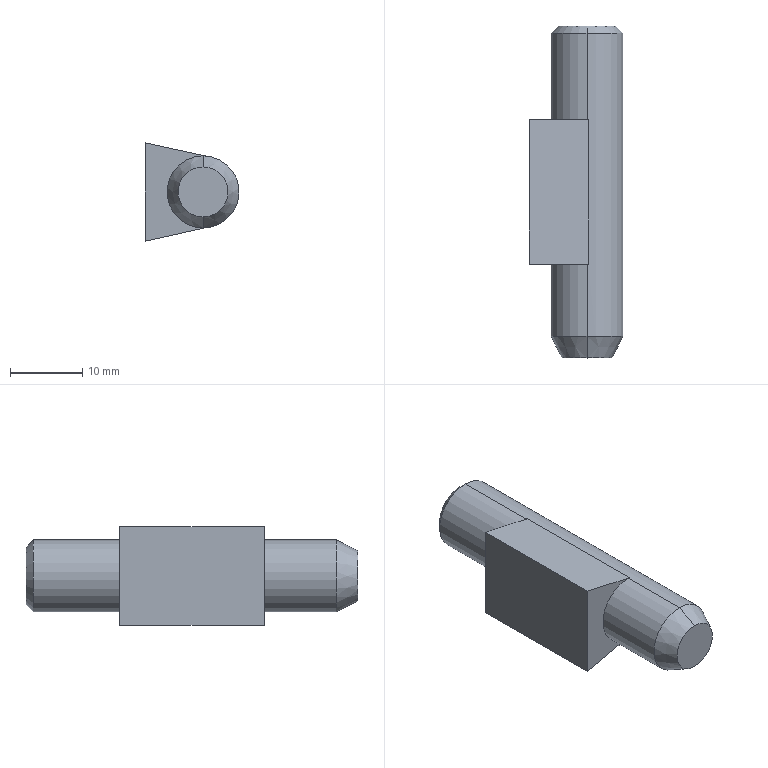Component | SolidWorks | Part21-1 | 1 solid | 20 faces | box 13.03 x 46 x 13.63 mm | volume 2575 mm3 | plane 9 | cylinder 7 | cone 4 | commonest cylinder face diameters 10 x3 8 x2 5.2 x2
STEP:
#1=COLOUR_RGB('',0.7922,0.8196,0.9333);
#2=FILL_AREA_STYLE_COLOUR('',#1);
#3=FILL_AREA_STYLE('',(#2));
#4=SURFACE_STYLE_FILL_AREA(#3);
#5=SURFACE_SIDE_STYLE('',(#4));
#6=SURFACE_STYLE_USAGE(.BOTH.,#5);
#7=PRESENTATION_STYLE_ASSIGNMENT((#6));
#8=CARTESIAN_POINT('',(6.044,10.866,-16.395));
#9=VERTEX_POINT('',#8);
#10=CARTESIAN_POINT('',(6.044,10.866,-16.08));
#11=VERTEX_POINT('',#10);
#12=CARTESIAN_POINT('',(6.044,10.866,-16.238));
#13=DIRECTION('',(0.,1.,0.));
#14=DIRECTION('',(0.,0.,-1.));
#15=AXIS2_PLACEMENT_3D('',#12,#13,#14);
#16=CIRCLE('',#15,0.1575);
#17=EDGE_CURVE('',#9,#11,#16,.T.);
#18=ORIENTED_EDGE('',*,*,#17,.F.);
#19=CARTESIAN_POINT('',(6.044,10.827,-16.434));
#20=VERTEX_POINT('',#19);
#21=CARTESIAN_POINT('',(6.044,10.866,-16.395));
#22=DIRECTION('',(-0.,-0.7071,-0.7071));
#23=VECTOR('',#22,39.37);
#24=LINE('',#21,#23);
#25=EDGE_CURVE('',#9,#20,#24,.T.);
#26=ORIENTED_EDGE('',*,*,#25,.T.);
#27=CARTESIAN_POINT('',(6.044,10.827,-16.041));
#28=VERTEX_POINT('',#27);
#29=CARTESIAN_POINT('',(6.044,10.827,-16.238));
#30=DIRECTION('',(-0.,-1.,-0.));
#31=DIRECTION('',(0.,0.,-1.));
#32=AXIS2_PLACEMENT_3D('',#29,#30,#31);
#33=CIRCLE('',#32,0.1969);
#34=EDGE_CURVE('',#28,#20,#33,.T.);
#35=ORIENTED_EDGE('',*,*,#34,.F.);
#36=CARTESIAN_POINT('',(6.044,10.866,-16.08));
#37=DIRECTION('',(-0.,-0.7071,0.7071));
#38=VECTOR('',#37,39.37);
#39=LINE('',#36,#38);
#40=EDGE_CURVE('',#11,#28,#39,.T.);
#41=ORIENTED_EDGE('',*,*,#40,.F.);
#42=EDGE_LOOP('',(#18,#26,#35,#41));
#43=FACE_OUTER_BOUND('',#42,.T.);
#44=CARTESIAN_POINT('',(6.044,10.866,-16.238));
#45=DIRECTION('',(-0.,-1.,-0.));
#46=DIRECTION('',(0.,0.,1.));
#47=AXIS2_PLACEMENT_3D('',#44,#45,#46);
#48=CONICAL_SURFACE('',#47,0.1575,0.7854);
#49=ADVANCED_FACE('',(#43),#48,.T.);
#50=CARTESIAN_POINT('',(6.044,10.748,-16.08));
#51=VERTEX_POINT('',#50);
#52=CARTESIAN_POINT('',(6.044,10.748,-16.395));
#53=VERTEX_POINT('',#52);
#54=CARTESIAN_POINT('',(6.044,10.748,-16.238));
#55=DIRECTION('',(0.,1.,0.));
#56=DIRECTION('',(0.,0.,-1.));
#57=AXIS2_PLACEMENT_3D('',#54,#55,#56);
#58=CIRCLE('',#57,0.1575);
#59=EDGE_CURVE('',#51,#53,#58,.T.);
#60=ORIENTED_EDGE('',*,*,#59,.T.);
#61=CARTESIAN_POINT('',(6.044,9.173,-16.395));
#62=VERTEX_POINT('',#61);
#63=CARTESIAN_POINT('',(6.044,10.748,-16.395));
#64=DIRECTION('',(-0.,-1.,-0.));
#65=VECTOR('',#64,39.37);
#66=LINE('',#63,#65);
#67=EDGE_CURVE('',#53,#62,#66,.T.);
#68=ORIENTED_EDGE('',*,*,#67,.T.);
#69=CARTESIAN_POINT('',(6.044,9.173,-16.08));
#70=VERTEX_POINT('',#69);
#71=CARTESIAN_POINT('',(6.044,9.173,-16.238));
#72=DIRECTION('',(0.,1.,0.));
#73=DIRECTION('',(0.,0.,-1.));
#74=AXIS2_PLACEMENT_3D('',#71,#72,#73);
#75=CIRCLE('',#74,0.1575);
#76=EDGE_CURVE('',#70,#62,#75,.T.);
#77=ORIENTED_EDGE('',*,*,#76,.F.);
#78=CARTESIAN_POINT('',(6.044,10.748,-16.08));
#79=DIRECTION('',(-0.,-1.,-0.));
#80=VECTOR('',#79,39.37);
#81=LINE('',#78,#80);
#82=EDGE_CURVE('',#51,#70,#81,.T.);
#83=ORIENTED_EDGE('',*,*,#82,.F.);
#84=EDGE_LOOP('',(#60,#68,#77,#83));
#85=FACE_OUTER_BOUND('',#84,.T.);
#86=CARTESIAN_POINT('',(6.044,10.748,-16.238));
#87=DIRECTION('',(-0.,-1.,-0.));
#88=DIRECTION('',(0.,0.,1.));
#89=AXIS2_PLACEMENT_3D('',#86,#87,#88);
#90=CYLINDRICAL_SURFACE('',#89,0.1575);
#91=ADVANCED_FACE('',(#85),#90,.F.);
#92=CARTESIAN_POINT('',(6.044,10.866,-16.135));
#93=VERTEX_POINT('',#92);
#94=CARTESIAN_POINT('',(6.044,10.866,-16.34));
#95=VERTEX_POINT('',#94);
#96=CARTESIAN_POINT('',(6.044,10.866,-16.238));
#97=DIRECTION('',(0.,1.,0.));
#98=DIRECTION('',(0.,0.,-1.));
#99=AXIS2_PLACEMENT_3D('',#96,#97,#98);
#100=CIRCLE('',#99,0.1024);
#101=EDGE_CURVE('',#93,#95,#100,.T.);
#102=ORIENTED_EDGE('',*,*,#101,.T.);
#103=CARTESIAN_POINT('',(6.044,10.748,-16.34));
#104=VERTEX_POINT('',#103);
#105=CARTESIAN_POINT('',(6.044,10.866,-16.34));
#106=DIRECTION('',(-0.,-1.,-0.));
#107=VECTOR('',#106,39.37);
#108=LINE('',#105,#107);
#109=EDGE_CURVE('',#95,#104,#108,.T.);
#110=ORIENTED_EDGE('',*,*,#109,.T.);
#111=CARTESIAN_POINT('',(6.044,10.748,-16.135));
#112=VERTEX_POINT('',#111);
#113=CARTESIAN_POINT('',(6.044,10.748,-16.238));
#114=DIRECTION('',(0.,1.,0.));
#115=DIRECTION('',(0.,0.,-1.));
#116=AXIS2_PLACEMENT_3D('',#113,#114,#115);
#117=CIRCLE('',#116,0.1024);
#118=EDGE_CURVE('',#112,#104,#117,.T.);
#119=ORIENTED_EDGE('',*,*,#118,.F.);
#120=CARTESIAN_POINT('',(6.044,10.866,-16.135));
#121=DIRECTION('',(-0.,-1.,-0.));
#122=VECTOR('',#121,39.37);
#123=LINE('',#120,#122);
#124=EDGE_CURVE('',#93,#112,#123,.T.);
#125=ORIENTED_EDGE('',*,*,#124,.F.);
#126=EDGE_LOOP('',(#102,#110,#119,#125));
#127=FACE_OUTER_BOUND('',#126,.T.);
#128=CARTESIAN_POINT('',(6.044,10.866,-16.238));
#129=DIRECTION('',(-0.,-1.,-0.));
#130=DIRECTION('',(0.,0.,1.));
#131=AXIS2_PLACEMENT_3D('',#128,#129,#130);
#132=CYLINDRICAL_SURFACE('',#131,0.1024);
#133=ADVANCED_FACE('',(#127),#132,.F.);
#134=CARTESIAN_POINT('',(6.044,9.055,-16.374));
#135=VERTEX_POINT('',#134);
#136=CARTESIAN_POINT('',(6.044,9.055,-16.101));
#137=VERTEX_POINT('',#136);
#138=CARTESIAN_POINT('',(6.044,9.055,-16.238));
#139=DIRECTION('',(-0.,-1.,-0.));
#140=DIRECTION('',(0.,0.,1.));
#141=AXIS2_PLACEMENT_3D('',#138,#139,#140);
#142=CIRCLE('',#141,0.1367);
#143=EDGE_CURVE('',#135,#137,#142,.T.);
#144=ORIENTED_EDGE('',*,*,#143,.F.);
#145=CARTESIAN_POINT('',(6.044,9.173,-16.434));
#146=VERTEX_POINT('',#145);
#147=CARTESIAN_POINT('',(6.044,9.173,-16.434));
#148=DIRECTION('',(0.,0.891,-0.454));
#149=VECTOR('',#148,39.37);
#150=LINE('',#147,#149);
#151=EDGE_CURVE('',#135,#146,#150,.T.);
#152=ORIENTED_EDGE('',*,*,#151,.T.);
#153=CARTESIAN_POINT('',(6.044,9.173,-16.041));
#154=VERTEX_POINT('',#153);
#155=CARTESIAN_POINT('',(6.044,9.173,-16.238));
#156=DIRECTION('',(-0.,-1.,-0.));
#157=DIRECTION('',(0.,0.,1.));
#158=AXIS2_PLACEMENT_3D('',#155,#156,#157);
#159=CIRCLE('',#158,0.1969);
#160=EDGE_CURVE('',#146,#154,#159,.T.);
#161=ORIENTED_EDGE('',*,*,#160,.T.);
#162=CARTESIAN_POINT('',(6.044,9.173,-16.041));
#163=DIRECTION('',(0.,0.891,0.454));
#164=VECTOR('',#163,39.37);
#165=LINE('',#162,#164);
#166=EDGE_CURVE('',#137,#154,#165,.T.);
#167=ORIENTED_EDGE('',*,*,#166,.F.);
#168=EDGE_LOOP('',(#144,#152,#161,#167));
#169=FACE_OUTER_BOUND('',#168,.T.);
#170=CARTESIAN_POINT('',(6.044,9.173,-16.238));
#171=DIRECTION('',(0.,1.,0.));
#172=DIRECTION('',(0.,0.,1.));
#173=AXIS2_PLACEMENT_3D('',#170,#171,#172);
#174=CONICAL_SURFACE('',#173,0.1969,0.4712);
#175=ADVANCED_FACE('',(#169),#174,.T.);
#176=ORIENTED_EDGE('',*,*,#34,.T.);
#177=CARTESIAN_POINT('',(6.044,10.354,-16.434));
#178=VERTEX_POINT('',#177);
#179=CARTESIAN_POINT('',(6.044,10.748,-16.434));
#180=DIRECTION('',(-0.,-1.,-0.));
#181=VECTOR('',#180,39.37);
#182=LINE('',#179,#181);
#183=EDGE_CURVE('',#20,#178,#182,.T.);
#184=ORIENTED_EDGE('',*,*,#183,.T.);
#185=CARTESIAN_POINT('',(6.044,10.354,-16.041));
#186=VERTEX_POINT('',#185);
#187=CARTESIAN_POINT('',(6.044,10.354,-16.238));
#188=DIRECTION('',(0.,1.,0.));
#189=DIRECTION('',(0.,0.,1.));
#190=AXIS2_PLACEMENT_3D('',#187,#188,#189);
#191=CIRCLE('',#190,0.1969);
#192=EDGE_CURVE('',#178,#186,#191,.T.);
#193=ORIENTED_EDGE('',*,*,#192,.T.);
#194=CARTESIAN_POINT('',(6.044,10.748,-16.041));
#195=DIRECTION('',(-0.,-1.,-0.));
#196=VECTOR('',#195,39.37);
#197=LINE('',#194,#196);
#198=EDGE_CURVE('',#28,#186,#197,.T.);
#199=ORIENTED_EDGE('',*,*,#198,.F.);
#200=EDGE_LOOP('',(#176,#184,#193,#199));
#201=FACE_OUTER_BOUND('',#200,.T.);
#202=CARTESIAN_POINT('',(6.044,10.748,-16.238));
#203=DIRECTION('',(-0.,-1.,-0.));
#204=DIRECTION('',(0.,0.,1.));
#205=AXIS2_PLACEMENT_3D('',#202,#203,#204);
#206=CYLINDRICAL_SURFACE('',#205,0.1969);
#207=ADVANCED_FACE('',(#201),#206,.T.);
#208=CARTESIAN_POINT('',(6.044,9.567,-16.434));
#209=VERTEX_POINT('',#208);
#210=CARTESIAN_POINT('',(6.044,9.567,-16.041));
#211=VERTEX_POINT('',#210);
#212=CARTESIAN_POINT('',(6.044,9.567,-16.238));
#213=DIRECTION('',(0.,1.,0.));
#214=DIRECTION('',(0.,0.,1.));
#215=AXIS2_PLACEMENT_3D('',#212,#213,#214);
#216=CIRCLE('',#215,0.1969);
#217=EDGE_CURVE('',#209,#211,#216,.T.);
#218=ORIENTED_EDGE('',*,*,#217,.F.);
#219=CARTESIAN_POINT('',(6.044,10.748,-16.434));
#220=DIRECTION('',(-0.,-1.,-0.));
#221=VECTOR('',#220,39.37);
#222=LINE('',#219,#221);
#223=EDGE_CURVE('',#209,#146,#222,.T.);
#224=ORIENTED_EDGE('',*,*,#223,.T.);
#225=CARTESIAN_POINT('',(6.044,9.173,-16.238));
#226=DIRECTION('',(-0.,-1.,-0.));
#227=DIRECTION('',(0.,0.,1.));
#228=AXIS2_PLACEMENT_3D('',#225,#226,#227);
#229=CIRCLE('',#228,0.1969);
#230=EDGE_CURVE('',#154,#146,#229,.T.);
#231=ORIENTED_EDGE('',*,*,#230,.F.);
#232=CARTESIAN_POINT('',(6.044,10.748,-16.041));
#233=DIRECTION('',(-0.,-1.,-0.));
#234=VECTOR('',#233,39.37);
#235=LINE('',#232,#234);
#236=EDGE_CURVE('',#211,#154,#235,.T.);
#237=ORIENTED_EDGE('',*,*,#236,.F.);
#238=EDGE_LOOP('',(#218,#224,#231,#237));
#239=FACE_OUTER_BOUND('',#238,.T.);
#240=CARTESIAN_POINT('',(6.044,10.748,-16.238));
#241=DIRECTION('',(-0.,-1.,-0.));
#242=DIRECTION('',(0.,0.,1.));
#243=AXIS2_PLACEMENT_3D('',#240,#241,#242);
#244=CYLINDRICAL_SURFACE('',#243,0.1969);
#245=ADVANCED_FACE('',(#239),#244,.T.);
#246=ORIENTED_EDGE('',*,*,#183,.F.);
#247=CARTESIAN_POINT('',(6.044,10.827,-16.238));
#248=DIRECTION('',(-0.,-1.,-0.));
#249=DIRECTION('',(0.,0.,-1.));
#250=AXIS2_PLACEMENT_3D('',#247,#248,#249);
#251=CIRCLE('',#250,0.1969);
#252=EDGE_CURVE('',#20,#28,#251,.T.);
#253=ORIENTED_EDGE('',*,*,#252,.T.);
#254=ORIENTED_EDGE('',*,*,#198,.T.);
#255=CARTESIAN_POINT('',(6.051,10.354,-16.041));
#256=VERTEX_POINT('',#255);
#257=CARTESIAN_POINT('',(6.044,10.354,-16.238));
#258=DIRECTION('',(0.,1.,0.));
#259=DIRECTION('',(0.,0.,1.));
#260=AXIS2_PLACEMENT_3D('',#257,#258,#259);
#261=CIRCLE('',#260,0.1969);
#262=EDGE_CURVE('',#186,#256,#261,.T.);
#263=ORIENTED_EDGE('',*,*,#262,.T.);
#264=CARTESIAN_POINT('',(6.051,9.567,-16.041));
#265=VERTEX_POINT('',#264);
#266=CARTESIAN_POINT('',(6.051,9.567,-16.041));
#267=DIRECTION('',(0.,1.,0.));
#268=VECTOR('',#267,39.37);
#269=LINE('',#266,#268);
#270=EDGE_CURVE('',#265,#256,#269,.T.);
#271=ORIENTED_EDGE('',*,*,#270,.F.);
#272=CARTESIAN_POINT('',(6.044,9.567,-16.238));
#273=DIRECTION('',(0.,1.,0.));
#274=DIRECTION('',(0.,0.,1.));
#275=AXIS2_PLACEMENT_3D('',#272,#273,#274);
#276=CIRCLE('',#275,0.1969);
#277=EDGE_CURVE('',#211,#265,#276,.T.);
#278=ORIENTED_EDGE('',*,*,#277,.F.);
#279=ORIENTED_EDGE('',*,*,#236,.T.);
#280=ORIENTED_EDGE('',*,*,#160,.F.);
#281=ORIENTED_EDGE('',*,*,#223,.F.);
#282=CARTESIAN_POINT('',(6.051,9.567,-16.434));
#283=VERTEX_POINT('',#282);
#284=CARTESIAN_POINT('',(6.044,9.567,-16.238));
#285=DIRECTION('',(0.,1.,0.));
#286=DIRECTION('',(0.,0.,1.));
#287=AXIS2_PLACEMENT_3D('',#284,#285,#286);
#288=CIRCLE('',#287,0.1969);
#289=EDGE_CURVE('',#283,#209,#288,.T.);
#290=ORIENTED_EDGE('',*,*,#289,.F.);
#291=CARTESIAN_POINT('',(6.051,10.354,-16.434));
#292=VERTEX_POINT('',#291);
#293=CARTESIAN_POINT('',(6.051,9.567,-16.434));
#294=DIRECTION('',(0.,1.,0.));
#295=VECTOR('',#294,39.37);
#296=LINE('',#293,#295);
#297=EDGE_CURVE('',#283,#292,#296,.T.);
#298=ORIENTED_EDGE('',*,*,#297,.T.);
#299=CARTESIAN_POINT('',(6.044,10.354,-16.238));
#300=DIRECTION('',(0.,1.,0.));
#301=DIRECTION('',(0.,0.,1.));
#302=AXIS2_PLACEMENT_3D('',#299,#300,#301);
#303=CIRCLE('',#302,0.1969);
#304=EDGE_CURVE('',#292,#178,#303,.T.);
#305=ORIENTED_EDGE('',*,*,#304,.T.);
#306=EDGE_LOOP('',(#246,#253,#254,#263,#271,#278,#279,#280,#281,#290,#298,#305));
#307=FACE_OUTER_BOUND('',#306,.T.);
#308=CARTESIAN_POINT('',(6.044,10.748,-16.238));
#309=DIRECTION('',(-0.,-1.,-0.));
#310=DIRECTION('',(0.,0.,1.));
#311=AXIS2_PLACEMENT_3D('',#308,#309,#310);
#312=CYLINDRICAL_SURFACE('',#311,0.1969);
#313=ADVANCED_FACE('',(#307),#312,.T.);
#314=ORIENTED_EDGE('',*,*,#151,.F.);
#315=CARTESIAN_POINT('',(6.044,9.055,-16.238));
#316=DIRECTION('',(-0.,-1.,-0.));
#317=DIRECTION('',(0.,0.,1.));
#318=AXIS2_PLACEMENT_3D('',#315,#316,#317);
#319=CIRCLE('',#318,0.1367);
#320=EDGE_CURVE('',#137,#135,#319,.T.);
#321=ORIENTED_EDGE('',*,*,#320,.F.);
#322=ORIENTED_EDGE('',*,*,#166,.T.);
#323=ORIENTED_EDGE('',*,*,#230,.T.);
#324=EDGE_LOOP('',(#314,#321,#322,#323));
#325=FACE_OUTER_BOUND('',#324,.T.);
#326=CARTESIAN_POINT('',(6.044,9.173,-16.238));
#327=DIRECTION('',(0.,1.,0.));
#328=DIRECTION('',(0.,0.,1.));
#329=AXIS2_PLACEMENT_3D('',#326,#327,#328);
#330=CONICAL_SURFACE('',#329,0.1969,0.4712);
#331=ADVANCED_FACE('',(#325),#330,.T.);
#332=ORIENTED_EDGE('',*,*,#320,.T.);
#333=ORIENTED_EDGE('',*,*,#143,.T.);
#334=EDGE_LOOP('',(#332,#333));
#335=FACE_OUTER_BOUND('',#334,.T.);
#336=CARTESIAN_POINT('',(6.044,9.055,-16.238));
#337=DIRECTION('',(-0.,-1.,-0.));
#338=DIRECTION('',(0.,-0.,1.));
#339=AXIS2_PLACEMENT_3D('',#336,#337,#338);
#340=PLANE('',#339);
#341=ADVANCED_FACE('',(#335),#340,.T.);
#342=ORIENTED_EDGE('',*,*,#270,.T.);
#343=CARTESIAN_POINT('',(5.728,10.354,-15.97));
#344=VERTEX_POINT('',#343);
#345=CARTESIAN_POINT('',(5.728,10.354,-15.97));
#346=DIRECTION('',(-0.9766,0.,0.2149));
#347=VECTOR('',#346,39.37);
#348=LINE('',#345,#347);
#349=EDGE_CURVE('',#256,#344,#348,.T.);
#350=ORIENTED_EDGE('',*,*,#349,.T.);
#351=CARTESIAN_POINT('',(5.728,9.567,-15.97));
#352=VERTEX_POINT('',#351);
#353=CARTESIAN_POINT('',(5.728,9.567,-15.97));
#354=DIRECTION('',(0.,1.,0.));
#355=VECTOR('',#354,39.37);
#356=LINE('',#353,#355);
#357=EDGE_CURVE('',#352,#344,#356,.T.);
#358=ORIENTED_EDGE('',*,*,#357,.F.);
#359=CARTESIAN_POINT('',(5.728,9.567,-15.97));
#360=DIRECTION('',(-0.9766,0.,0.2149));
#361=VECTOR('',#360,39.37);
#362=LINE('',#359,#361);
#363=EDGE_CURVE('',#265,#352,#362,.T.);
#364=ORIENTED_EDGE('',*,*,#363,.F.);
#365=EDGE_LOOP('',(#342,#350,#358,#364));
#366=FACE_OUTER_BOUND('',#365,.T.);
#367=CARTESIAN_POINT('',(5.728,9.567,-15.97));
#368=DIRECTION('',(-0.2149,0.,-0.9766));
#369=DIRECTION('',(-0.9766,0.,0.2149));
#370=AXIS2_PLACEMENT_3D('',#367,#368,#369);
#371=PLANE('',#370);
#372=ADVANCED_FACE('',(#366),#371,.F.);
#373=ORIENTED_EDGE('',*,*,#357,.T.);
#374=CARTESIAN_POINT('',(5.728,10.354,-16.506));
#375=VERTEX_POINT('',#374);
#376=CARTESIAN_POINT('',(5.728,10.354,-16.506));
#377=DIRECTION('',(-0.,0.,-1.));
#378=VECTOR('',#377,39.37);
#379=LINE('',#376,#378);
#380=EDGE_CURVE('',#344,#375,#379,.T.);
#381=ORIENTED_EDGE('',*,*,#380,.T.);
#382=CARTESIAN_POINT('',(5.728,9.567,-16.506));
#383=VERTEX_POINT('',#382);
#384=CARTESIAN_POINT('',(5.728,9.567,-16.506));
#385=DIRECTION('',(0.,1.,0.));
#386=VECTOR('',#385,39.37);
#387=LINE('',#384,#386);
#388=EDGE_CURVE('',#383,#375,#387,.T.);
#389=ORIENTED_EDGE('',*,*,#388,.F.);
#390=CARTESIAN_POINT('',(5.728,9.567,-16.506));
#391=DIRECTION('',(-0.,0.,-1.));
#392=VECTOR('',#391,39.37);
#393=LINE('',#390,#392);
#394=EDGE_CURVE('',#352,#383,#393,.T.);
#395=ORIENTED_EDGE('',*,*,#394,.F.);
#396=EDGE_LOOP('',(#373,#381,#389,#395));
#397=FACE_OUTER_BOUND('',#396,.T.);
#398=CARTESIAN_POINT('',(5.728,9.567,-16.506));
#399=DIRECTION('',(1.,-0.,-0.));
#400=DIRECTION('',(-0.,-1.,-0.));
#401=AXIS2_PLACEMENT_3D('',#398,#399,#400);
#402=PLANE('',#401);
#403=ADVANCED_FACE('',(#397),#402,.F.);
#404=ORIENTED_EDGE('',*,*,#388,.T.);
#405=CARTESIAN_POINT('',(6.051,10.354,-16.434));
#406=DIRECTION('',(0.9759,-0.,0.218));
#407=VECTOR('',#406,39.37);
#408=LINE('',#405,#407);
#409=EDGE_CURVE('',#375,#292,#408,.T.);
#410=ORIENTED_EDGE('',*,*,#409,.T.);
#411=ORIENTED_EDGE('',*,*,#297,.F.);
#412=CARTESIAN_POINT('',(6.051,9.567,-16.434));
#413=DIRECTION('',(0.9759,-0.,0.218));
#414=VECTOR('',#413,39.37);
#415=LINE('',#412,#414);
#416=EDGE_CURVE('',#383,#283,#415,.T.);
#417=ORIENTED_EDGE('',*,*,#416,.F.);
#418=EDGE_LOOP('',(#404,#410,#411,#417));
#419=FACE_OUTER_BOUND('',#418,.T.);
#420=CARTESIAN_POINT('',(6.051,9.567,-16.434));
#421=DIRECTION('',(-0.218,0.,0.9759));
#422=DIRECTION('',(0.9759,-0.,0.218));
#423=AXIS2_PLACEMENT_3D('',#420,#421,#422);
#424=PLANE('',#423);
#425=ADVANCED_FACE('',(#419),#424,.F.);
#426=ORIENTED_EDGE('',*,*,#289,.T.);
#427=ORIENTED_EDGE('',*,*,#217,.T.);
#428=ORIENTED_EDGE('',*,*,#277,.T.);
#429=ORIENTED_EDGE('',*,*,#363,.T.);
#430=ORIENTED_EDGE('',*,*,#394,.T.);
#431=ORIENTED_EDGE('',*,*,#416,.T.);
#432=EDGE_LOOP('',(#426,#427,#428,#429,#430,#431));
#433=FACE_OUTER_BOUND('',#432,.T.);
#434=CARTESIAN_POINT('',(6.044,9.567,-16.238));
#435=DIRECTION('',(-0.,-1.,-0.));
#436=DIRECTION('',(0.,-0.,1.));
#437=AXIS2_PLACEMENT_3D('',#434,#435,#436);
#438=PLANE('',#437);
#439=ADVANCED_FACE('',(#433),#438,.T.);
#440=ORIENTED_EDGE('',*,*,#304,.F.);
#441=ORIENTED_EDGE('',*,*,#409,.F.);
#442=ORIENTED_EDGE('',*,*,#380,.F.);
#443=ORIENTED_EDGE('',*,*,#349,.F.);
#444=ORIENTED_EDGE('',*,*,#262,.F.);
#445=ORIENTED_EDGE('',*,*,#192,.F.);
#446=EDGE_LOOP('',(#440,#441,#442,#443,#444,#445));
#447=FACE_OUTER_BOUND('',#446,.T.);
#448=CARTESIAN_POINT('',(6.044,10.354,-16.238));
#449=DIRECTION('',(-0.,-1.,-0.));
#450=DIRECTION('',(0.,-0.,1.));
#451=AXIS2_PLACEMENT_3D('',#448,#449,#450);
#452=PLANE('',#451);
#453=ADVANCED_FACE('',(#447),#452,.F.);
#454=ORIENTED_EDGE('',*,*,#118,.T.);
#455=CARTESIAN_POINT('',(6.044,10.748,-16.238));
#456=DIRECTION('',(0.,1.,0.));
#457=DIRECTION('',(0.,0.,-1.));
#458=AXIS2_PLACEMENT_3D('',#455,#456,#457);
#459=CIRCLE('',#458,0.1024);
#460=EDGE_CURVE('',#104,#112,#459,.T.);
#461=ORIENTED_EDGE('',*,*,#460,.T.);
#462=EDGE_LOOP('',(#454,#461));
#463=FACE_BOUND('',#462,.T.);
#464=ORIENTED_EDGE('',*,*,#59,.F.);
#465=CARTESIAN_POINT('',(6.044,10.748,-16.238));
#466=DIRECTION('',(0.,1.,0.));
#467=DIRECTION('',(0.,0.,-1.));
#468=AXIS2_PLACEMENT_3D('',#465,#466,#467);
#469=CIRCLE('',#468,0.1575);
#470=EDGE_CURVE('',#53,#51,#469,.T.);
#471=ORIENTED_EDGE('',*,*,#470,.F.);
#472=EDGE_LOOP('',(#464,#471));
#473=FACE_OUTER_BOUND('',#472,.T.);
#474=CARTESIAN_POINT('',(6.044,10.748,-16.238));
#475=DIRECTION('',(0.,1.,0.));
#476=DIRECTION('',(-0.,0.,-1.));
#477=AXIS2_PLACEMENT_3D('',#474,#475,#476);
#478=PLANE('',#477);
#479=ADVANCED_FACE('',(#463,#473),#478,.F.);
#480=CARTESIAN_POINT('',(6.044,10.866,-16.238));
#481=DIRECTION('',(0.,1.,0.));
#482=DIRECTION('',(0.,0.,-1.));
#483=AXIS2_PLACEMENT_3D('',#480,#481,#482);
#484=CIRCLE('',#483,0.1575);
#485=EDGE_CURVE('',#11,#9,#484,.T.);
#486=ORIENTED_EDGE('',*,*,#485,.T.);
#487=ORIENTED_EDGE('',*,*,#17,.T.);
#488=EDGE_LOOP('',(#486,#487));
#489=FACE_OUTER_BOUND('',#488,.T.);
#490=ORIENTED_EDGE('',*,*,#101,.F.);
#491=CARTESIAN_POINT('',(6.044,10.866,-16.238));
#492=DIRECTION('',(0.,1.,0.));
#493=DIRECTION('',(0.,0.,-1.));
#494=AXIS2_PLACEMENT_3D('',#491,#492,#493);
#495=CIRCLE('',#494,0.1024);
#496=EDGE_CURVE('',#95,#93,#495,.T.);
#497=ORIENTED_EDGE('',*,*,#496,.F.);
#498=EDGE_LOOP('',(#490,#497));
#499=FACE_BOUND('',#498,.T.);
#500=CARTESIAN_POINT('',(6.044,10.866,-16.238));
#501=DIRECTION('',(0.,1.,0.));
#502=DIRECTION('',(-0.,0.,-1.));
#503=AXIS2_PLACEMENT_3D('',#500,#501,#502);
#504=PLANE('',#503);
#505=ADVANCED_FACE('',(#489,#499),#504,.T.);
#506=ORIENTED_EDGE('',*,*,#109,.F.);
#507=ORIENTED_EDGE('',*,*,#496,.T.);
#508=ORIENTED_EDGE('',*,*,#124,.T.);
#509=ORIENTED_EDGE('',*,*,#460,.F.);
#510=EDGE_LOOP('',(#506,#507,#508,#509));
#511=FACE_OUTER_BOUND('',#510,.T.);
#512=CARTESIAN_POINT('',(6.044,10.866,-16.238));
#513=DIRECTION('',(-0.,-1.,-0.));
#514=DIRECTION('',(0.,0.,1.));
#515=AXIS2_PLACEMENT_3D('',#512,#513,#514);
#516=CYLINDRICAL_SURFACE('',#515,0.1024);
#517=ADVANCED_FACE('',(#511),#516,.F.);
#518=ORIENTED_EDGE('',*,*,#76,.T.);
#519=CARTESIAN_POINT('',(6.044,9.173,-16.238));
#520=DIRECTION('',(0.,1.,0.));
#521=DIRECTION('',(0.,0.,-1.));
#522=AXIS2_PLACEMENT_3D('',#519,#520,#521);
#523=CIRCLE('',#522,0.1575);
#524=EDGE_CURVE('',#62,#70,#523,.T.);
#525=ORIENTED_EDGE('',*,*,#524,.T.);
#526=EDGE_LOOP('',(#518,#525));
#527=FACE_OUTER_BOUND('',#526,.T.);
#528=CARTESIAN_POINT('',(6.044,9.173,-16.238));
#529=DIRECTION('',(-0.,-1.,-0.));
#530=DIRECTION('',(0.,-0.,1.));
#531=AXIS2_PLACEMENT_3D('',#528,#529,#530);
#532=PLANE('',#531);
#533=ADVANCED_FACE('',(#527),#532,.F.);
#534=ORIENTED_EDGE('',*,*,#67,.F.);
#535=ORIENTED_EDGE('',*,*,#470,.T.);
#536=ORIENTED_EDGE('',*,*,#82,.T.);
#537=ORIENTED_EDGE('',*,*,#524,.F.);
#538=EDGE_LOOP('',(#534,#535,#536,#537));
#539=FACE_OUTER_BOUND('',#538,.T.);
#540=CARTESIAN_POINT('',(6.044,10.748,-16.238));
#541=DIRECTION('',(-0.,-1.,-0.));
#542=DIRECTION('',(0.,0.,1.));
#543=AXIS2_PLACEMENT_3D('',#540,#541,#542);
#544=CYLINDRICAL_SURFACE('',#543,0.1575);
#545=ADVANCED_FACE('',(#539),#544,.F.);
#546=ORIENTED_EDGE('',*,*,#25,.F.);
#547=ORIENTED_EDGE('',*,*,#485,.F.);
#548=ORIENTED_EDGE('',*,*,#40,.T.);
#549=ORIENTED_EDGE('',*,*,#252,.F.);
#550=EDGE_LOOP('',(#546,#547,#548,#549));
#551=FACE_OUTER_BOUND('',#550,.T.);
#552=CARTESIAN_POINT('',(6.044,10.866,-16.238));
#553=DIRECTION('',(-0.,-1.,-0.));
#554=DIRECTION('',(0.,0.,1.));
#555=AXIS2_PLACEMENT_3D('',#552,#553,#554);
#556=CONICAL_SURFACE('',#555,0.1575,0.7854);
#557=ADVANCED_FACE('',(#551),#556,.T.);
#558=CLOSED_SHELL('',(#49,#91,#133,#175,#207,#245,#313,#331,#341,#372,#403,#425,#439,#453,#479,#505,#517,#533,#545,#557));
#559=MANIFOLD_SOLID_BREP('',#558);
#560=STYLED_ITEM('',(#7),#559);
#561=(LENGTH_UNIT()NAMED_UNIT(*)SI_UNIT($,.METRE.));
#562=LENGTH_MEASURE_WITH_UNIT(LENGTH_MEASURE(0.0254),#561);
#563=DIMENSIONAL_EXPONENTS(1.,0.,0.,0.,0.,0.,0.);
#564=(CONVERSION_BASED_UNIT('',#562)LENGTH_UNIT()NAMED_UNIT(#563));
#565=UNCERTAINTY_MEASURE_WITH_UNIT(LENGTH_MEASURE(0.00001),#564,'','');
#566=(NAMED_UNIT(*)PLANE_ANGLE_UNIT()SI_UNIT($,.RADIAN.));
#567=(NAMED_UNIT(*)SI_UNIT($,.STERADIAN.)SOLID_ANGLE_UNIT());
#568=(GEOMETRIC_REPRESENTATION_CONTEXT(3)GLOBAL_UNCERTAINTY_ASSIGNED_CONTEXT((#565))GLOBAL_UNIT_ASSIGNED_CONTEXT((#564,#566,#567))REPRESENTATION_CONTEXT('',''));
#569=MECHANICAL_DESIGN_GEOMETRIC_PRESENTATION_REPRESENTATION('',(#560),#568);
#570=CARTESIAN_POINT('',(0.,0.,0.));
#571=DIRECTION('',(0.,0.,1.));
#572=DIRECTION('',(1.,0.,0.));
#573=AXIS2_PLACEMENT_3D('',#570,#571,#572);
#574=(LENGTH_UNIT()NAMED_UNIT(*)SI_UNIT($,.METRE.));
#575=LENGTH_MEASURE_WITH_UNIT(LENGTH_MEASURE(0.0254),#574);
#576=DIMENSIONAL_EXPONENTS(1.,0.,0.,0.,0.,0.,0.);
#577=(CONVERSION_BASED_UNIT('',#575)LENGTH_UNIT()NAMED_UNIT(#576));
#578=UNCERTAINTY_MEASURE_WITH_UNIT(LENGTH_MEASURE(0.00001),#577,'','');
#579=(NAMED_UNIT(*)PLANE_ANGLE_UNIT()SI_UNIT($,.RADIAN.));
#580=(NAMED_UNIT(*)SI_UNIT($,.STERADIAN.)SOLID_ANGLE_UNIT());
#581=(GEOMETRIC_REPRESENTATION_CONTEXT(3)GLOBAL_UNCERTAINTY_ASSIGNED_CONTEXT((#578))GLOBAL_UNIT_ASSIGNED_CONTEXT((#577,#579,#580))REPRESENTATION_CONTEXT('',''));
#582=ADVANCED_BREP_SHAPE_REPRESENTATION('',(#559,#573),#581);
#583=PRESENTATION_LAYER_ASSIGNMENT('','',(#560));